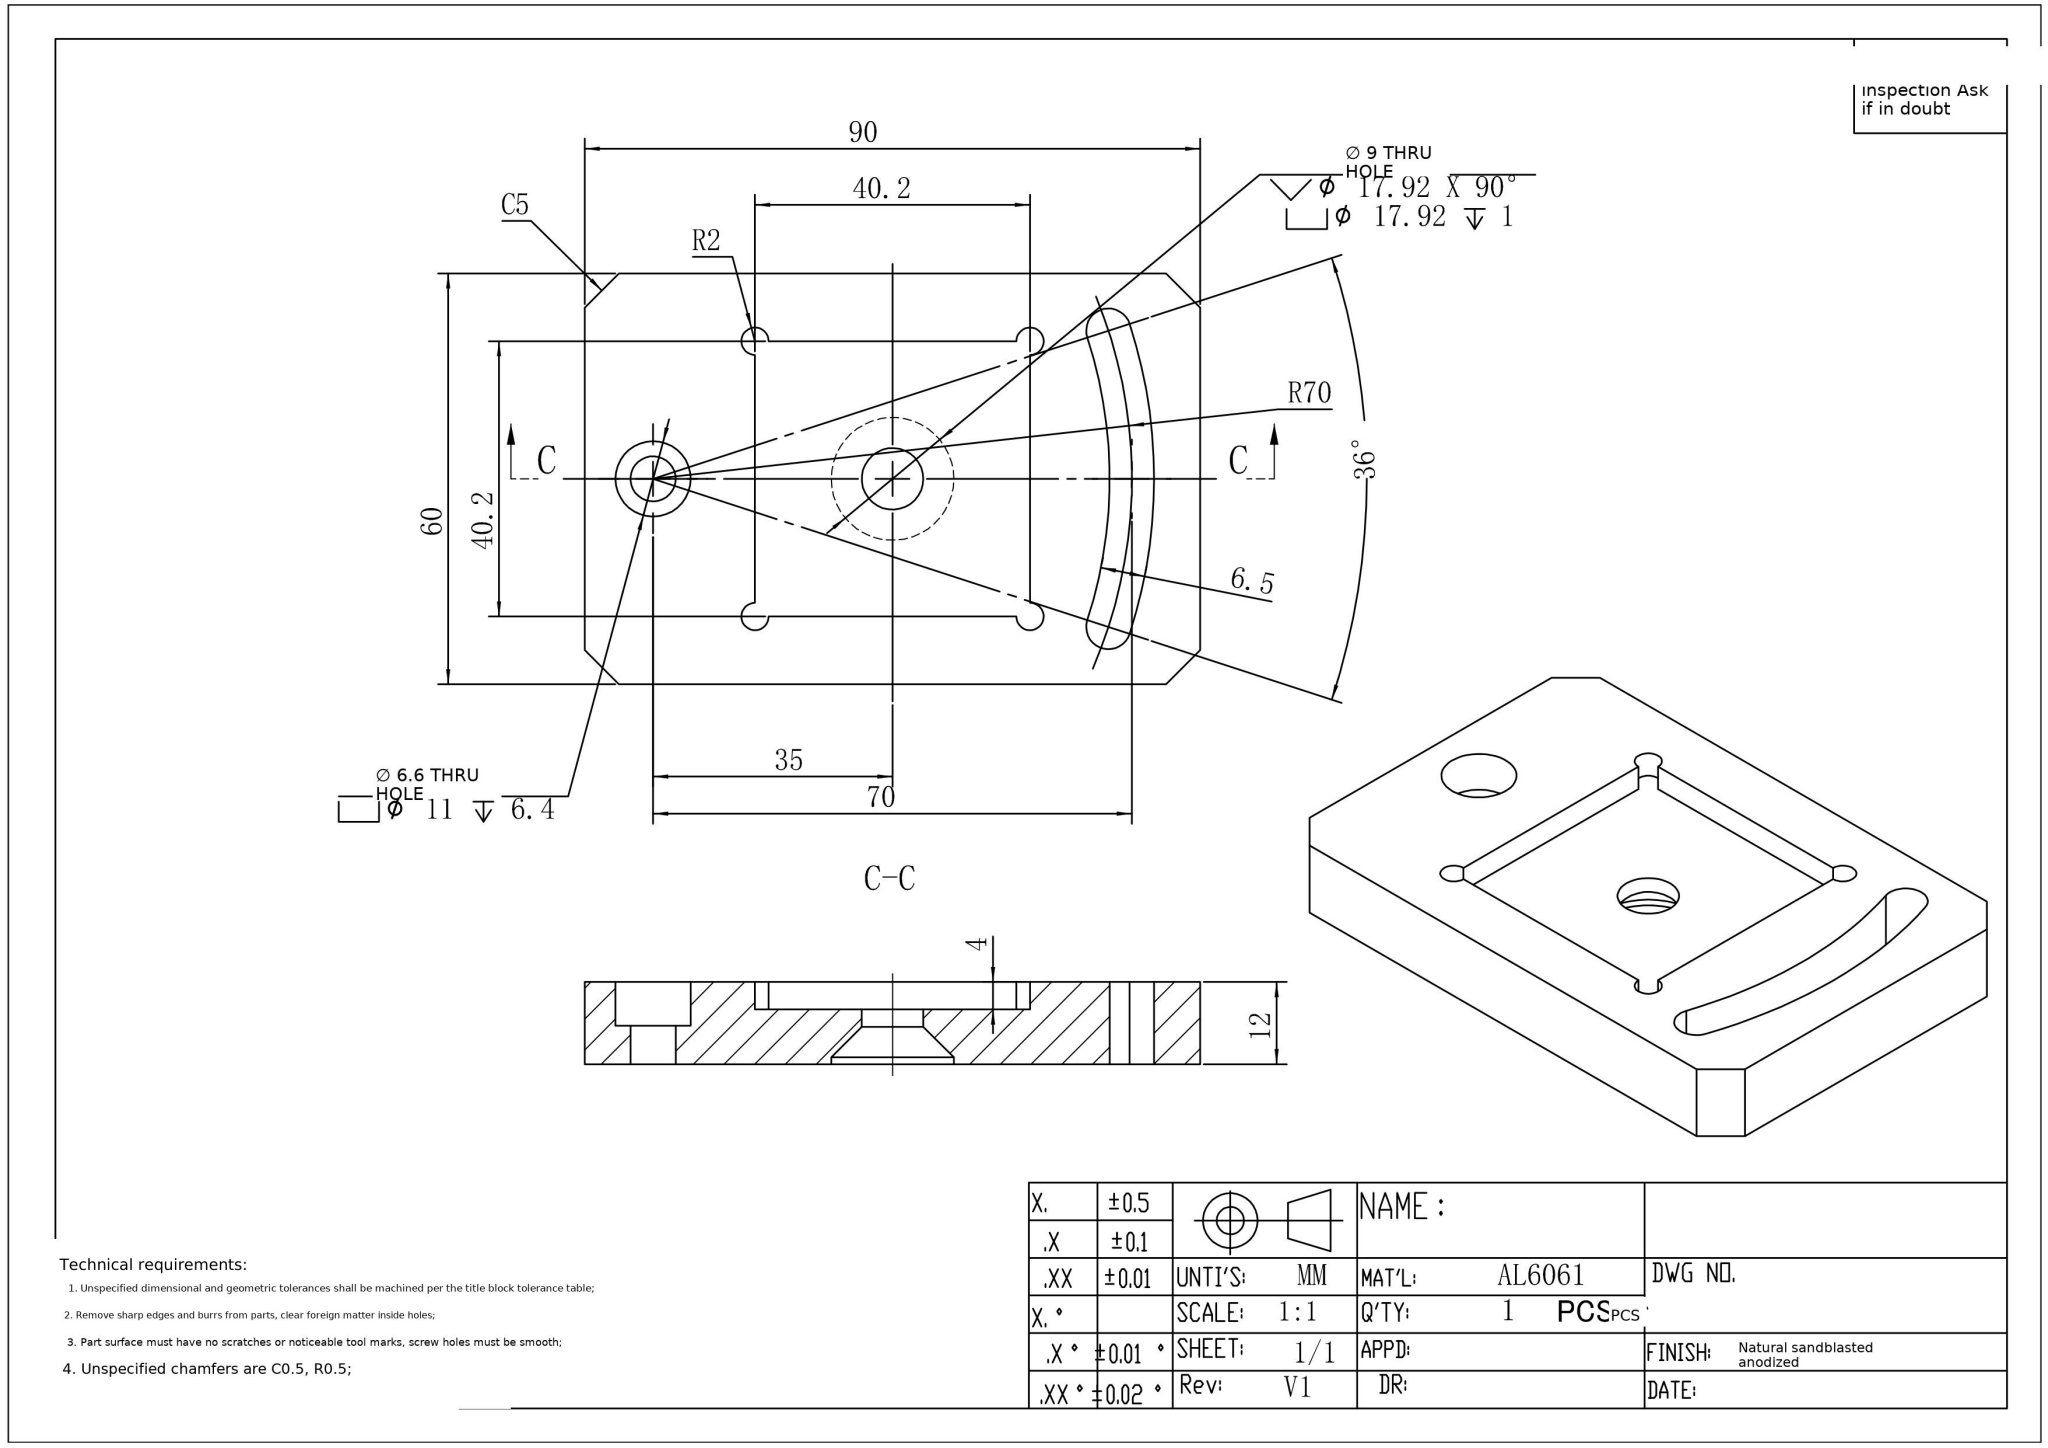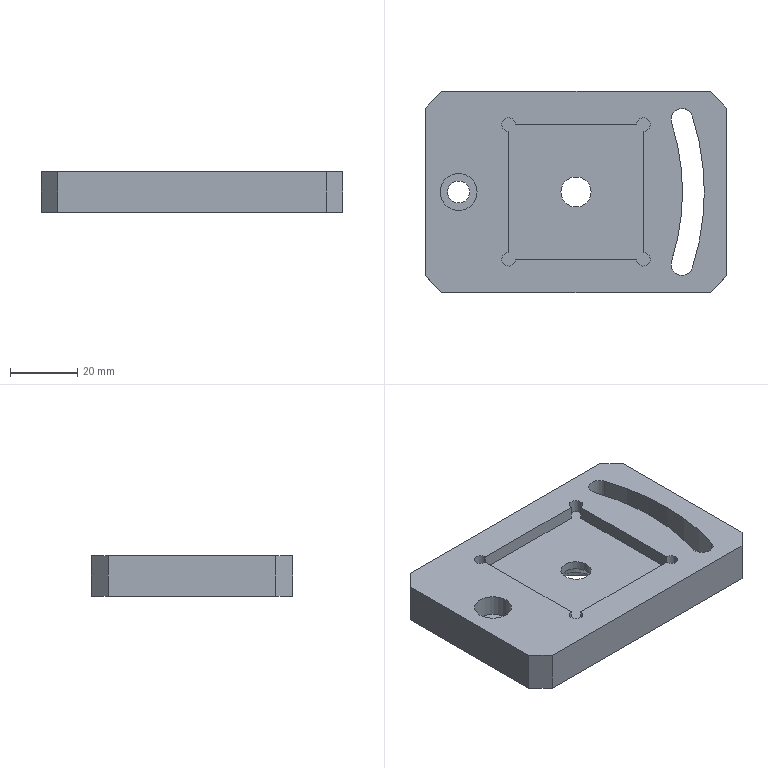Part | NX | mm | 1 solid | 29 faces | box 90 x 60 x 12 mm | volume 51885 mm3 | plane 16 | cylinder 12 | cone 1 | commonest cylinder face diameters 4 x4 6.5 x2 6.6 x1 11 x1 133.5 x1 146.5 x1 17.92 x1 9 x1
STEP:
#1=CARTESIAN_POINT('',(0.,0.,0.));
#2=DIRECTION('',(0.,0.,1.));
#3=DIRECTION('',(1.,0.,0.));
#4=AXIS2_PLACEMENT_3D('',#1,#2,#3);
#5=(LENGTH_UNIT()NAMED_UNIT(*)SI_UNIT(.MILLI.,.METRE.));
#6=UNCERTAINTY_MEASURE_WITH_UNIT(LENGTH_MEASURE(0.00002),#5,'','');
#7=(NAMED_UNIT(*)PLANE_ANGLE_UNIT()SI_UNIT($,.RADIAN.));
#8=PLANE_ANGLE_MEASURE_WITH_UNIT(PLANE_ANGLE_MEASURE(0.01745),#7);
#9=DIMENSIONAL_EXPONENTS(0.,0.,0.,0.,0.,0.,0.);
#10=(CONVERSION_BASED_UNIT('',#8)NAMED_UNIT(#9)PLANE_ANGLE_UNIT());
#11=(NAMED_UNIT(*)SI_UNIT($,.STERADIAN.)SOLID_ANGLE_UNIT());
#12=(GEOMETRIC_REPRESENTATION_CONTEXT(3)GLOBAL_UNCERTAINTY_ASSIGNED_CONTEXT((#6))GLOBAL_UNIT_ASSIGNED_CONTEXT((#5,#10,#11))REPRESENTATION_CONTEXT('',''));
#13=SHAPE_REPRESENTATION('',(#4),#12);
#14=CARTESIAN_POINT('',(85.,60.,0.));
#15=VERTEX_POINT('',#14);
#16=CARTESIAN_POINT('',(5.,60.,0.));
#17=VERTEX_POINT('',#16);
#18=CARTESIAN_POINT('',(90.,60.,0.));
#19=DIRECTION('',(-1.,0.,0.));
#20=VECTOR('',#19,1.);
#21=LINE('',#18,#20);
#22=EDGE_CURVE('',#15,#17,#21,.T.);
#23=ORIENTED_EDGE('',*,*,#22,.F.);
#24=CARTESIAN_POINT('',(85.,60.,-12.));
#25=VERTEX_POINT('',#24);
#26=CARTESIAN_POINT('',(85.,60.,-12.));
#27=DIRECTION('',(0.,0.,-1.));
#28=VECTOR('',#27,1.);
#29=LINE('',#26,#28);
#30=EDGE_CURVE('',#15,#25,#29,.T.);
#31=ORIENTED_EDGE('',*,*,#30,.T.);
#32=CARTESIAN_POINT('',(5.,60.,-12.));
#33=VERTEX_POINT('',#32);
#34=CARTESIAN_POINT('',(90.,60.,-12.));
#35=DIRECTION('',(-1.,0.,0.));
#36=VECTOR('',#35,1.);
#37=LINE('',#34,#36);
#38=EDGE_CURVE('',#25,#33,#37,.T.);
#39=ORIENTED_EDGE('',*,*,#38,.T.);
#40=CARTESIAN_POINT('',(5.,60.,-12.));
#41=DIRECTION('',(0.,0.,1.));
#42=VECTOR('',#41,1.);
#43=LINE('',#40,#42);
#44=EDGE_CURVE('',#33,#17,#43,.T.);
#45=ORIENTED_EDGE('',*,*,#44,.T.);
#46=EDGE_LOOP('',(#23,#31,#39,#45));
#47=FACE_OUTER_BOUND('',#46,.T.);
#48=CARTESIAN_POINT('',(90.,60.,-12.));
#49=DIRECTION('',(0.,1.,0.));
#50=DIRECTION('',(0.,0.,1.));
#51=AXIS2_PLACEMENT_3D('',#48,#49,#50);
#52=PLANE('',#51);
#53=ADVANCED_FACE('',(#47),#52,.T.);
#54=CARTESIAN_POINT('',(0.,55.,-12.));
#55=VERTEX_POINT('',#54);
#56=CARTESIAN_POINT('',(0.,5.,-12.));
#57=VERTEX_POINT('',#56);
#58=CARTESIAN_POINT('',(0.,60.,-12.));
#59=DIRECTION('',(0.,-1.,0.));
#60=VECTOR('',#59,1.);
#61=LINE('',#58,#60);
#62=EDGE_CURVE('',#55,#57,#61,.T.);
#63=ORIENTED_EDGE('',*,*,#62,.T.);
#64=CARTESIAN_POINT('',(0.,5.,0.));
#65=VERTEX_POINT('',#64);
#66=CARTESIAN_POINT('',(0.,5.,-12.));
#67=DIRECTION('',(0.,0.,1.));
#68=VECTOR('',#67,1.);
#69=LINE('',#66,#68);
#70=EDGE_CURVE('',#57,#65,#69,.T.);
#71=ORIENTED_EDGE('',*,*,#70,.T.);
#72=CARTESIAN_POINT('',(0.,55.,0.));
#73=VERTEX_POINT('',#72);
#74=CARTESIAN_POINT('',(0.,60.,0.));
#75=DIRECTION('',(0.,-1.,0.));
#76=VECTOR('',#75,1.);
#77=LINE('',#74,#76);
#78=EDGE_CURVE('',#73,#65,#77,.T.);
#79=ORIENTED_EDGE('',*,*,#78,.F.);
#80=CARTESIAN_POINT('',(0.,55.,-12.));
#81=DIRECTION('',(0.,0.,-1.));
#82=VECTOR('',#81,1.);
#83=LINE('',#80,#82);
#84=EDGE_CURVE('',#73,#55,#83,.T.);
#85=ORIENTED_EDGE('',*,*,#84,.T.);
#86=EDGE_LOOP('',(#63,#71,#79,#85));
#87=FACE_OUTER_BOUND('',#86,.T.);
#88=CARTESIAN_POINT('',(0.,60.,-12.));
#89=DIRECTION('',(-1.,0.,0.));
#90=DIRECTION('',(0.,0.,1.));
#91=AXIS2_PLACEMENT_3D('',#88,#89,#90);
#92=PLANE('',#91);
#93=ADVANCED_FACE('',(#87),#92,.T.);
#94=CARTESIAN_POINT('',(5.,0.,0.));
#95=VERTEX_POINT('',#94);
#96=CARTESIAN_POINT('',(85.,0.,0.));
#97=VERTEX_POINT('',#96);
#98=CARTESIAN_POINT('',(0.,0.,0.));
#99=DIRECTION('',(1.,-0.,0.));
#100=VECTOR('',#99,1.);
#101=LINE('',#98,#100);
#102=EDGE_CURVE('',#95,#97,#101,.T.);
#103=ORIENTED_EDGE('',*,*,#102,.F.);
#104=CARTESIAN_POINT('',(5.,0.,-12.));
#105=VERTEX_POINT('',#104);
#106=CARTESIAN_POINT('',(5.,0.,-12.));
#107=DIRECTION('',(0.,0.,-1.));
#108=VECTOR('',#107,1.);
#109=LINE('',#106,#108);
#110=EDGE_CURVE('',#95,#105,#109,.T.);
#111=ORIENTED_EDGE('',*,*,#110,.T.);
#112=CARTESIAN_POINT('',(85.,0.,-12.));
#113=VERTEX_POINT('',#112);
#114=CARTESIAN_POINT('',(0.,0.,-12.));
#115=DIRECTION('',(1.,-0.,0.));
#116=VECTOR('',#115,1.);
#117=LINE('',#114,#116);
#118=EDGE_CURVE('',#105,#113,#117,.T.);
#119=ORIENTED_EDGE('',*,*,#118,.T.);
#120=CARTESIAN_POINT('',(85.,0.,-12.));
#121=DIRECTION('',(0.,0.,1.));
#122=VECTOR('',#121,1.);
#123=LINE('',#120,#122);
#124=EDGE_CURVE('',#113,#97,#123,.T.);
#125=ORIENTED_EDGE('',*,*,#124,.T.);
#126=EDGE_LOOP('',(#103,#111,#119,#125));
#127=FACE_OUTER_BOUND('',#126,.T.);
#128=CARTESIAN_POINT('',(0.,0.,-12.));
#129=DIRECTION('',(-0.,-1.,0.));
#130=DIRECTION('',(1.,-0.,0.));
#131=AXIS2_PLACEMENT_3D('',#128,#129,#130);
#132=PLANE('',#131);
#133=ADVANCED_FACE('',(#127),#132,.T.);
#134=CARTESIAN_POINT('',(90.,5.,0.));
#135=VERTEX_POINT('',#134);
#136=CARTESIAN_POINT('',(90.,55.,0.));
#137=VERTEX_POINT('',#136);
#138=CARTESIAN_POINT('',(90.,0.,0.));
#139=DIRECTION('',(-0.,1.,0.));
#140=VECTOR('',#139,1.);
#141=LINE('',#138,#140);
#142=EDGE_CURVE('',#135,#137,#141,.T.);
#143=ORIENTED_EDGE('',*,*,#142,.F.);
#144=CARTESIAN_POINT('',(90.,5.,-12.));
#145=VERTEX_POINT('',#144);
#146=CARTESIAN_POINT('',(90.,5.,-12.));
#147=DIRECTION('',(0.,0.,-1.));
#148=VECTOR('',#147,1.);
#149=LINE('',#146,#148);
#150=EDGE_CURVE('',#135,#145,#149,.T.);
#151=ORIENTED_EDGE('',*,*,#150,.T.);
#152=CARTESIAN_POINT('',(90.,55.,-12.));
#153=VERTEX_POINT('',#152);
#154=CARTESIAN_POINT('',(90.,0.,-12.));
#155=DIRECTION('',(-0.,1.,0.));
#156=VECTOR('',#155,1.);
#157=LINE('',#154,#156);
#158=EDGE_CURVE('',#145,#153,#157,.T.);
#159=ORIENTED_EDGE('',*,*,#158,.T.);
#160=CARTESIAN_POINT('',(90.,55.,-12.));
#161=DIRECTION('',(0.,0.,1.));
#162=VECTOR('',#161,1.);
#163=LINE('',#160,#162);
#164=EDGE_CURVE('',#153,#137,#163,.T.);
#165=ORIENTED_EDGE('',*,*,#164,.T.);
#166=EDGE_LOOP('',(#143,#151,#159,#165));
#167=FACE_OUTER_BOUND('',#166,.T.);
#168=CARTESIAN_POINT('',(90.,0.,-12.));
#169=DIRECTION('',(1.,0.,0.));
#170=DIRECTION('',(-0.,1.,0.));
#171=AXIS2_PLACEMENT_3D('',#168,#169,#170);
#172=PLANE('',#171);
#173=ADVANCED_FACE('',(#167),#172,.T.);
#174=CARTESIAN_POINT('',(53.96,30.,-12.));
#175=VERTEX_POINT('',#174);
#176=CARTESIAN_POINT('',(45.,30.,-12.));
#177=DIRECTION('',(0.,0.,1.));
#178=DIRECTION('',(1.,0.,0.));
#179=AXIS2_PLACEMENT_3D('',#176,#177,#178);
#180=CIRCLE('',#179,8.96);
#181=EDGE_CURVE('',#175,#175,#180,.T.);
#182=ORIENTED_EDGE('',*,*,#181,.T.);
#183=EDGE_LOOP('',(#182));
#184=FACE_BOUND('',#183,.T.);
#185=CARTESIAN_POINT('',(79.665,7.365,-12.));
#186=VERTEX_POINT('',#185);
#187=CARTESIAN_POINT('',(73.483,9.373,-12.));
#188=VERTEX_POINT('',#187);
#189=CARTESIAN_POINT('',(76.574,8.369,-12.));
#190=DIRECTION('',(0.,0.,-1.));
#191=DIRECTION('',(1.,0.,0.));
#192=AXIS2_PLACEMENT_3D('',#189,#190,#191);
#193=CIRCLE('',#192,3.25);
#194=EDGE_CURVE('',#186,#188,#193,.T.);
#195=ORIENTED_EDGE('',*,*,#194,.F.);
#196=CARTESIAN_POINT('',(79.665,52.635,-12.));
#197=VERTEX_POINT('',#196);
#198=CARTESIAN_POINT('',(10.,30.,-12.));
#199=DIRECTION('',(0.,0.,-1.));
#200=DIRECTION('',(1.,0.,0.));
#201=AXIS2_PLACEMENT_3D('',#198,#199,#200);
#202=CIRCLE('',#201,73.25);
#203=EDGE_CURVE('',#197,#186,#202,.T.);
#204=ORIENTED_EDGE('',*,*,#203,.F.);
#205=CARTESIAN_POINT('',(73.483,50.627,-12.));
#206=VERTEX_POINT('',#205);
#207=CARTESIAN_POINT('',(76.574,51.631,-12.));
#208=DIRECTION('',(0.,0.,-1.));
#209=DIRECTION('',(1.,0.,0.));
#210=AXIS2_PLACEMENT_3D('',#207,#208,#209);
#211=CIRCLE('',#210,3.25);
#212=EDGE_CURVE('',#206,#197,#211,.T.);
#213=ORIENTED_EDGE('',*,*,#212,.F.);
#214=CARTESIAN_POINT('',(10.,30.,-12.));
#215=DIRECTION('',(0.,0.,1.));
#216=DIRECTION('',(1.,0.,0.));
#217=AXIS2_PLACEMENT_3D('',#214,#215,#216);
#218=CIRCLE('',#217,66.75);
#219=EDGE_CURVE('',#188,#206,#218,.T.);
#220=ORIENTED_EDGE('',*,*,#219,.F.);
#221=EDGE_LOOP('',(#195,#204,#213,#220));
#222=FACE_BOUND('',#221,.T.);
#223=CARTESIAN_POINT('',(13.3,30.,-12.));
#224=VERTEX_POINT('',#223);
#225=CARTESIAN_POINT('',(10.,30.,-12.));
#226=DIRECTION('',(0.,0.,1.));
#227=DIRECTION('',(1.,0.,0.));
#228=AXIS2_PLACEMENT_3D('',#225,#226,#227);
#229=CIRCLE('',#228,3.3);
#230=EDGE_CURVE('',#224,#224,#229,.T.);
#231=ORIENTED_EDGE('',*,*,#230,.T.);
#232=EDGE_LOOP('',(#231));
#233=FACE_BOUND('',#232,.T.);
#234=ORIENTED_EDGE('',*,*,#118,.F.);
#235=CARTESIAN_POINT('',(0.,5.,-12.));
#236=DIRECTION('',(-0.7071,0.7071,0.));
#237=VECTOR('',#236,1.);
#238=LINE('',#235,#237);
#239=EDGE_CURVE('',#105,#57,#238,.T.);
#240=ORIENTED_EDGE('',*,*,#239,.T.);
#241=ORIENTED_EDGE('',*,*,#62,.F.);
#242=CARTESIAN_POINT('',(5.,60.,-12.));
#243=DIRECTION('',(0.7071,0.7071,0.));
#244=VECTOR('',#243,1.);
#245=LINE('',#242,#244);
#246=EDGE_CURVE('',#55,#33,#245,.T.);
#247=ORIENTED_EDGE('',*,*,#246,.T.);
#248=ORIENTED_EDGE('',*,*,#38,.F.);
#249=CARTESIAN_POINT('',(90.,55.,-12.));
#250=DIRECTION('',(0.7071,-0.7071,0.));
#251=VECTOR('',#250,1.);
#252=LINE('',#249,#251);
#253=EDGE_CURVE('',#25,#153,#252,.T.);
#254=ORIENTED_EDGE('',*,*,#253,.T.);
#255=ORIENTED_EDGE('',*,*,#158,.F.);
#256=CARTESIAN_POINT('',(85.,0.,-12.));
#257=DIRECTION('',(-0.7071,-0.7071,0.));
#258=VECTOR('',#257,1.);
#259=LINE('',#256,#258);
#260=EDGE_CURVE('',#145,#113,#259,.T.);
#261=ORIENTED_EDGE('',*,*,#260,.T.);
#262=EDGE_LOOP('',(#234,#240,#241,#247,#248,#254,#255,#261));
#263=FACE_BOUND('',#262,.T.);
#264=CARTESIAN_POINT('',(0.,0.,-12.));
#265=DIRECTION('',(0.,0.,1.));
#266=DIRECTION('',(1.,0.,0.));
#267=AXIS2_PLACEMENT_3D('',#264,#265,#266);
#268=PLANE('',#267);
#269=ADVANCED_FACE('',(#184,#222,#233,#263),#268,.F.);
#270=CARTESIAN_POINT('',(79.665,52.635,0.));
#271=VERTEX_POINT('',#270);
#272=CARTESIAN_POINT('',(79.665,7.365,0.));
#273=VERTEX_POINT('',#272);
#274=CARTESIAN_POINT('',(10.,30.,0.));
#275=DIRECTION('',(0.,0.,-1.));
#276=DIRECTION('',(1.,0.,0.));
#277=AXIS2_PLACEMENT_3D('',#274,#275,#276);
#278=CIRCLE('',#277,73.25);
#279=EDGE_CURVE('',#271,#273,#278,.T.);
#280=ORIENTED_EDGE('',*,*,#279,.T.);
#281=CARTESIAN_POINT('',(73.483,9.373,0.));
#282=VERTEX_POINT('',#281);
#283=CARTESIAN_POINT('',(76.574,8.369,0.));
#284=DIRECTION('',(0.,0.,-1.));
#285=DIRECTION('',(1.,0.,0.));
#286=AXIS2_PLACEMENT_3D('',#283,#284,#285);
#287=CIRCLE('',#286,3.25);
#288=EDGE_CURVE('',#273,#282,#287,.T.);
#289=ORIENTED_EDGE('',*,*,#288,.T.);
#290=CARTESIAN_POINT('',(73.483,50.627,0.));
#291=VERTEX_POINT('',#290);
#292=CARTESIAN_POINT('',(10.,30.,0.));
#293=DIRECTION('',(0.,0.,1.));
#294=DIRECTION('',(1.,0.,0.));
#295=AXIS2_PLACEMENT_3D('',#292,#293,#294);
#296=CIRCLE('',#295,66.75);
#297=EDGE_CURVE('',#282,#291,#296,.T.);
#298=ORIENTED_EDGE('',*,*,#297,.T.);
#299=CARTESIAN_POINT('',(76.574,51.631,0.));
#300=DIRECTION('',(0.,0.,-1.));
#301=DIRECTION('',(1.,0.,0.));
#302=AXIS2_PLACEMENT_3D('',#299,#300,#301);
#303=CIRCLE('',#302,3.25);
#304=EDGE_CURVE('',#291,#271,#303,.T.);
#305=ORIENTED_EDGE('',*,*,#304,.T.);
#306=EDGE_LOOP('',(#280,#289,#298,#305));
#307=FACE_BOUND('',#306,.T.);
#308=CARTESIAN_POINT('',(65.1,11.9,0.));
#309=VERTEX_POINT('',#308);
#310=CARTESIAN_POINT('',(65.1,48.1,0.));
#311=VERTEX_POINT('',#310);
#312=CARTESIAN_POINT('',(65.1,11.9,0.));
#313=DIRECTION('',(0.,1.,0.));
#314=VECTOR('',#313,1.);
#315=LINE('',#312,#314);
#316=EDGE_CURVE('',#309,#311,#315,.T.);
#317=ORIENTED_EDGE('',*,*,#316,.F.);
#318=CARTESIAN_POINT('',(63.1,9.9,0.));
#319=VERTEX_POINT('',#318);
#320=CARTESIAN_POINT('',(65.1,9.9,0.));
#321=DIRECTION('',(0.,0.,1.));
#322=DIRECTION('',(1.,0.,0.));
#323=AXIS2_PLACEMENT_3D('',#320,#321,#322);
#324=CIRCLE('',#323,2.);
#325=EDGE_CURVE('',#319,#309,#324,.T.);
#326=ORIENTED_EDGE('',*,*,#325,.F.);
#327=CARTESIAN_POINT('',(26.9,9.9,0.));
#328=VERTEX_POINT('',#327);
#329=CARTESIAN_POINT('',(26.9,9.9,0.));
#330=DIRECTION('',(1.,0.,0.));
#331=VECTOR('',#330,1.);
#332=LINE('',#329,#331);
#333=EDGE_CURVE('',#328,#319,#332,.T.);
#334=ORIENTED_EDGE('',*,*,#333,.F.);
#335=CARTESIAN_POINT('',(24.9,11.9,0.));
#336=VERTEX_POINT('',#335);
#337=CARTESIAN_POINT('',(24.9,9.9,0.));
#338=DIRECTION('',(0.,0.,1.));
#339=DIRECTION('',(1.,0.,0.));
#340=AXIS2_PLACEMENT_3D('',#337,#338,#339);
#341=CIRCLE('',#340,2.);
#342=EDGE_CURVE('',#336,#328,#341,.T.);
#343=ORIENTED_EDGE('',*,*,#342,.F.);
#344=CARTESIAN_POINT('',(24.9,48.1,0.));
#345=VERTEX_POINT('',#344);
#346=CARTESIAN_POINT('',(24.9,48.1,0.));
#347=DIRECTION('',(0.,-1.,0.));
#348=VECTOR('',#347,1.);
#349=LINE('',#346,#348);
#350=EDGE_CURVE('',#345,#336,#349,.T.);
#351=ORIENTED_EDGE('',*,*,#350,.F.);
#352=CARTESIAN_POINT('',(26.9,50.1,0.));
#353=VERTEX_POINT('',#352);
#354=CARTESIAN_POINT('',(24.9,50.1,0.));
#355=DIRECTION('',(0.,0.,1.));
#356=DIRECTION('',(1.,0.,0.));
#357=AXIS2_PLACEMENT_3D('',#354,#355,#356);
#358=CIRCLE('',#357,2.);
#359=EDGE_CURVE('',#353,#345,#358,.T.);
#360=ORIENTED_EDGE('',*,*,#359,.F.);
#361=CARTESIAN_POINT('',(63.1,50.1,0.));
#362=VERTEX_POINT('',#361);
#363=CARTESIAN_POINT('',(63.1,50.1,0.));
#364=DIRECTION('',(-1.,0.,0.));
#365=VECTOR('',#364,1.);
#366=LINE('',#363,#365);
#367=EDGE_CURVE('',#362,#353,#366,.T.);
#368=ORIENTED_EDGE('',*,*,#367,.F.);
#369=CARTESIAN_POINT('',(65.1,50.1,0.));
#370=DIRECTION('',(0.,0.,1.));
#371=DIRECTION('',(1.,0.,0.));
#372=AXIS2_PLACEMENT_3D('',#369,#370,#371);
#373=CIRCLE('',#372,2.);
#374=EDGE_CURVE('',#311,#362,#373,.T.);
#375=ORIENTED_EDGE('',*,*,#374,.F.);
#376=EDGE_LOOP('',(#317,#326,#334,#343,#351,#360,#368,#375));
#377=FACE_BOUND('',#376,.T.);
#378=CARTESIAN_POINT('',(15.5,30.,0.));
#379=VERTEX_POINT('',#378);
#380=CARTESIAN_POINT('',(10.,30.,0.));
#381=DIRECTION('',(0.,0.,-1.));
#382=DIRECTION('',(1.,0.,0.));
#383=AXIS2_PLACEMENT_3D('',#380,#381,#382);
#384=CIRCLE('',#383,5.5);
#385=EDGE_CURVE('',#379,#379,#384,.T.);
#386=ORIENTED_EDGE('',*,*,#385,.T.);
#387=EDGE_LOOP('',(#386));
#388=FACE_BOUND('',#387,.T.);
#389=ORIENTED_EDGE('',*,*,#78,.T.);
#390=CARTESIAN_POINT('',(2.5,2.5,0.));
#391=DIRECTION('',(0.7071,-0.7071,0.));
#392=VECTOR('',#391,1.);
#393=LINE('',#390,#392);
#394=EDGE_CURVE('',#65,#95,#393,.T.);
#395=ORIENTED_EDGE('',*,*,#394,.T.);
#396=ORIENTED_EDGE('',*,*,#102,.T.);
#397=CARTESIAN_POINT('',(42.5,-42.5,0.));
#398=DIRECTION('',(0.7071,0.7071,0.));
#399=VECTOR('',#398,1.);
#400=LINE('',#397,#399);
#401=EDGE_CURVE('',#97,#135,#400,.T.);
#402=ORIENTED_EDGE('',*,*,#401,.T.);
#403=ORIENTED_EDGE('',*,*,#142,.T.);
#404=CARTESIAN_POINT('',(72.5,72.5,0.));
#405=DIRECTION('',(-0.7071,0.7071,0.));
#406=VECTOR('',#405,1.);
#407=LINE('',#404,#406);
#408=EDGE_CURVE('',#137,#15,#407,.T.);
#409=ORIENTED_EDGE('',*,*,#408,.T.);
#410=ORIENTED_EDGE('',*,*,#22,.T.);
#411=CARTESIAN_POINT('',(-27.5,27.5,0.));
#412=DIRECTION('',(-0.7071,-0.7071,0.));
#413=VECTOR('',#412,1.);
#414=LINE('',#411,#413);
#415=EDGE_CURVE('',#17,#73,#414,.T.);
#416=ORIENTED_EDGE('',*,*,#415,.T.);
#417=EDGE_LOOP('',(#389,#395,#396,#402,#403,#409,#410,#416));
#418=FACE_BOUND('',#417,.T.);
#419=CARTESIAN_POINT('',(0.,0.,0.));
#420=DIRECTION('',(0.,0.,1.));
#421=DIRECTION('',(1.,0.,0.));
#422=AXIS2_PLACEMENT_3D('',#419,#420,#421);
#423=PLANE('',#422);
#424=ADVANCED_FACE('',(#307,#377,#388,#418),#423,.T.);
#425=CARTESIAN_POINT('',(6.7,30.,-6.4));
#426=VERTEX_POINT('',#425);
#427=CARTESIAN_POINT('',(10.,30.,-6.4));
#428=DIRECTION('',(0.,0.,1.));
#429=DIRECTION('',(-1.,0.,0.));
#430=AXIS2_PLACEMENT_3D('',#427,#428,#429);
#431=CIRCLE('',#430,3.3);
#432=EDGE_CURVE('',#426,#426,#431,.T.);
#433=ORIENTED_EDGE('',*,*,#432,.T.);
#434=EDGE_LOOP('',(#433));
#435=FACE_BOUND('',#434,.T.);
#436=ORIENTED_EDGE('',*,*,#230,.F.);
#437=EDGE_LOOP('',(#436));
#438=FACE_BOUND('',#437,.T.);
#439=CARTESIAN_POINT('',(10.,30.,-12.));
#440=DIRECTION('',(0.,0.,1.));
#441=DIRECTION('',(1.,0.,0.));
#442=AXIS2_PLACEMENT_3D('',#439,#440,#441);
#443=CYLINDRICAL_SURFACE('',#442,3.3);
#444=ADVANCED_FACE('',(#435,#438),#443,.F.);
#445=CARTESIAN_POINT('',(15.5,30.,-6.4));
#446=VERTEX_POINT('',#445);
#447=CARTESIAN_POINT('',(10.,30.,-6.4));
#448=DIRECTION('',(0.,0.,1.));
#449=DIRECTION('',(1.,0.,0.));
#450=AXIS2_PLACEMENT_3D('',#447,#448,#449);
#451=CIRCLE('',#450,5.5);
#452=EDGE_CURVE('',#446,#446,#451,.T.);
#453=ORIENTED_EDGE('',*,*,#452,.T.);
#454=EDGE_LOOP('',(#453));
#455=FACE_BOUND('',#454,.T.);
#456=ORIENTED_EDGE('',*,*,#432,.F.);
#457=EDGE_LOOP('',(#456));
#458=FACE_BOUND('',#457,.T.);
#459=CARTESIAN_POINT('',(10.,30.,-6.4));
#460=DIRECTION('',(0.,0.,-1.));
#461=DIRECTION('',(-1.,0.,0.));
#462=AXIS2_PLACEMENT_3D('',#459,#460,#461);
#463=PLANE('',#462);
#464=ADVANCED_FACE('',(#455,#458),#463,.F.);
#465=ORIENTED_EDGE('',*,*,#452,.F.);
#466=EDGE_LOOP('',(#465));
#467=FACE_BOUND('',#466,.T.);
#468=ORIENTED_EDGE('',*,*,#385,.F.);
#469=EDGE_LOOP('',(#468));
#470=FACE_BOUND('',#469,.T.);
#471=CARTESIAN_POINT('',(10.,30.,-6.4));
#472=DIRECTION('',(0.,0.,1.));
#473=DIRECTION('',(1.,0.,0.));
#474=AXIS2_PLACEMENT_3D('',#471,#472,#473);
#475=CYLINDRICAL_SURFACE('',#474,5.5);
#476=ADVANCED_FACE('',(#467,#470),#475,.F.);
#477=ORIENTED_EDGE('',*,*,#316,.T.);
#478=CARTESIAN_POINT('',(65.1,48.1,-4.));
#479=VERTEX_POINT('',#478);
#480=CARTESIAN_POINT('',(65.1,48.1,-4.));
#481=DIRECTION('',(0.,0.,-1.));
#482=VECTOR('',#481,1.);
#483=LINE('',#480,#482);
#484=EDGE_CURVE('',#311,#479,#483,.T.);
#485=ORIENTED_EDGE('',*,*,#484,.T.);
#486=CARTESIAN_POINT('',(65.1,11.9,-4.));
#487=VERTEX_POINT('',#486);
#488=CARTESIAN_POINT('',(65.1,11.9,-4.));
#489=DIRECTION('',(0.,-1.,0.));
#490=VECTOR('',#489,1.);
#491=LINE('',#488,#490);
#492=EDGE_CURVE('',#479,#487,#491,.T.);
#493=ORIENTED_EDGE('',*,*,#492,.T.);
#494=CARTESIAN_POINT('',(65.1,11.9,-4.));
#495=DIRECTION('',(0.,0.,-1.));
#496=VECTOR('',#495,1.);
#497=LINE('',#494,#496);
#498=EDGE_CURVE('',#309,#487,#497,.T.);
#499=ORIENTED_EDGE('',*,*,#498,.F.);
#500=EDGE_LOOP('',(#477,#485,#493,#499));
#501=FACE_OUTER_BOUND('',#500,.T.);
#502=CARTESIAN_POINT('',(65.1,11.9,-4.));
#503=DIRECTION('',(1.,0.,0.));
#504=DIRECTION('',(0.,0.,-1.));
#505=AXIS2_PLACEMENT_3D('',#502,#503,#504);
#506=PLANE('',#505);
#507=ADVANCED_FACE('',(#501),#506,.F.);
#508=ORIENTED_EDGE('',*,*,#374,.T.);
#509=CARTESIAN_POINT('',(63.1,50.1,-4.));
#510=VERTEX_POINT('',#509);
#511=CARTESIAN_POINT('',(63.1,50.1,-4.));
#512=DIRECTION('',(0.,0.,-1.));
#513=VECTOR('',#512,1.);
#514=LINE('',#511,#513);
#515=EDGE_CURVE('',#362,#510,#514,.T.);
#516=ORIENTED_EDGE('',*,*,#515,.T.);
#517=CARTESIAN_POINT('',(65.1,50.1,-4.));
#518=DIRECTION('',(0.,0.,-1.));
#519=DIRECTION('',(1.,0.,0.));
#520=AXIS2_PLACEMENT_3D('',#517,#518,#519);
#521=CIRCLE('',#520,2.);
#522=EDGE_CURVE('',#510,#479,#521,.T.);
#523=ORIENTED_EDGE('',*,*,#522,.T.);
#524=ORIENTED_EDGE('',*,*,#484,.F.);
#525=EDGE_LOOP('',(#508,#516,#523,#524));
#526=FACE_OUTER_BOUND('',#525,.T.);
#527=CARTESIAN_POINT('',(65.1,50.1,-4.));
#528=DIRECTION('',(0.,0.,1.));
#529=DIRECTION('',(1.,0.,0.));
#530=AXIS2_PLACEMENT_3D('',#527,#528,#529);
#531=CYLINDRICAL_SURFACE('',#530,2.);
#532=ADVANCED_FACE('',(#526),#531,.F.);
#533=ORIENTED_EDGE('',*,*,#367,.T.);
#534=CARTESIAN_POINT('',(26.9,50.1,-4.));
#535=VERTEX_POINT('',#534);
#536=CARTESIAN_POINT('',(26.9,50.1,-4.));
#537=DIRECTION('',(0.,0.,-1.));
#538=VECTOR('',#537,1.);
#539=LINE('',#536,#538);
#540=EDGE_CURVE('',#353,#535,#539,.T.);
#541=ORIENTED_EDGE('',*,*,#540,.T.);
#542=CARTESIAN_POINT('',(63.1,50.1,-4.));
#543=DIRECTION('',(1.,0.,0.));
#544=VECTOR('',#543,1.);
#545=LINE('',#542,#544);
#546=EDGE_CURVE('',#535,#510,#545,.T.);
#547=ORIENTED_EDGE('',*,*,#546,.T.);
#548=ORIENTED_EDGE('',*,*,#515,.F.);
#549=EDGE_LOOP('',(#533,#541,#547,#548));
#550=FACE_OUTER_BOUND('',#549,.T.);
#551=CARTESIAN_POINT('',(63.1,50.1,-4.));
#552=DIRECTION('',(0.,1.,0.));
#553=DIRECTION('',(0.,0.,1.));
#554=AXIS2_PLACEMENT_3D('',#551,#552,#553);
#555=PLANE('',#554);
#556=ADVANCED_FACE('',(#550),#555,.F.);
#557=ORIENTED_EDGE('',*,*,#359,.T.);
#558=CARTESIAN_POINT('',(24.9,48.1,-4.));
#559=VERTEX_POINT('',#558);
#560=CARTESIAN_POINT('',(24.9,48.1,-4.));
#561=DIRECTION('',(0.,0.,-1.));
#562=VECTOR('',#561,1.);
#563=LINE('',#560,#562);
#564=EDGE_CURVE('',#345,#559,#563,.T.);
#565=ORIENTED_EDGE('',*,*,#564,.T.);
#566=CARTESIAN_POINT('',(24.9,50.1,-4.));
#567=DIRECTION('',(0.,0.,-1.));
#568=DIRECTION('',(1.,0.,0.));
#569=AXIS2_PLACEMENT_3D('',#566,#567,#568);
#570=CIRCLE('',#569,2.);
#571=EDGE_CURVE('',#559,#535,#570,.T.);
#572=ORIENTED_EDGE('',*,*,#571,.T.);
#573=ORIENTED_EDGE('',*,*,#540,.F.);
#574=EDGE_LOOP('',(#557,#565,#572,#573));
#575=FACE_OUTER_BOUND('',#574,.T.);
#576=CARTESIAN_POINT('',(24.9,50.1,-4.));
#577=DIRECTION('',(0.,0.,1.));
#578=DIRECTION('',(1.,0.,0.));
#579=AXIS2_PLACEMENT_3D('',#576,#577,#578);
#580=CYLINDRICAL_SURFACE('',#579,2.);
#581=ADVANCED_FACE('',(#575),#580,.F.);
#582=ORIENTED_EDGE('',*,*,#350,.T.);
#583=CARTESIAN_POINT('',(24.9,11.9,-4.));
#584=VERTEX_POINT('',#583);
#585=CARTESIAN_POINT('',(24.9,11.9,-4.));
#586=DIRECTION('',(0.,0.,-1.));
#587=VECTOR('',#586,1.);
#588=LINE('',#585,#587);
#589=EDGE_CURVE('',#336,#584,#588,.T.);
#590=ORIENTED_EDGE('',*,*,#589,.T.);
#591=CARTESIAN_POINT('',(24.9,48.1,-4.));
#592=DIRECTION('',(0.,1.,0.));
#593=VECTOR('',#592,1.);
#594=LINE('',#591,#593);
#595=EDGE_CURVE('',#584,#559,#594,.T.);
#596=ORIENTED_EDGE('',*,*,#595,.T.);
#597=ORIENTED_EDGE('',*,*,#564,.F.);
#598=EDGE_LOOP('',(#582,#590,#596,#597));
#599=FACE_OUTER_BOUND('',#598,.T.);
#600=CARTESIAN_POINT('',(24.9,48.1,-4.));
#601=DIRECTION('',(-1.,0.,0.));
#602=DIRECTION('',(0.,0.,1.));
#603=AXIS2_PLACEMENT_3D('',#600,#601,#602);
#604=PLANE('',#603);
#605=ADVANCED_FACE('',(#599),#604,.F.);
#606=ORIENTED_EDGE('',*,*,#342,.T.);
#607=CARTESIAN_POINT('',(26.9,9.9,-4.));
#608=VERTEX_POINT('',#607);
#609=CARTESIAN_POINT('',(26.9,9.9,-4.));
#610=DIRECTION('',(0.,0.,-1.));
#611=VECTOR('',#610,1.);
#612=LINE('',#609,#611);
#613=EDGE_CURVE('',#328,#608,#612,.T.);
#614=ORIENTED_EDGE('',*,*,#613,.T.);
#615=CARTESIAN_POINT('',(24.9,9.9,-4.));
#616=DIRECTION('',(0.,0.,-1.));
#617=DIRECTION('',(1.,0.,0.));
#618=AXIS2_PLACEMENT_3D('',#615,#616,#617);
#619=CIRCLE('',#618,2.);
#620=EDGE_CURVE('',#608,#584,#619,.T.);
#621=ORIENTED_EDGE('',*,*,#620,.T.);
#622=ORIENTED_EDGE('',*,*,#589,.F.);
#623=EDGE_LOOP('',(#606,#614,#621,#622));
#624=FACE_OUTER_BOUND('',#623,.T.);
#625=CARTESIAN_POINT('',(24.9,9.9,-4.));
#626=DIRECTION('',(0.,0.,1.));
#627=DIRECTION('',(1.,0.,0.));
#628=AXIS2_PLACEMENT_3D('',#625,#626,#627);
#629=CYLINDRICAL_SURFACE('',#628,2.);
#630=ADVANCED_FACE('',(#624),#629,.F.);
#631=ORIENTED_EDGE('',*,*,#333,.T.);
#632=CARTESIAN_POINT('',(63.1,9.9,-4.));
#633=VERTEX_POINT('',#632);
#634=CARTESIAN_POINT('',(63.1,9.9,-4.));
#635=DIRECTION('',(0.,0.,-1.));
#636=VECTOR('',#635,1.);
#637=LINE('',#634,#636);
#638=EDGE_CURVE('',#319,#633,#637,.T.);
#639=ORIENTED_EDGE('',*,*,#638,.T.);
#640=CARTESIAN_POINT('',(26.9,9.9,-4.));
#641=DIRECTION('',(-1.,0.,0.));
#642=VECTOR('',#641,1.);
#643=LINE('',#640,#642);
#644=EDGE_CURVE('',#633,#608,#643,.T.);
#645=ORIENTED_EDGE('',*,*,#644,.T.);
#646=ORIENTED_EDGE('',*,*,#613,.F.);
#647=EDGE_LOOP('',(#631,#639,#645,#646));
#648=FACE_OUTER_BOUND('',#647,.T.);
#649=CARTESIAN_POINT('',(26.9,9.9,-4.));
#650=DIRECTION('',(0.,-1.,0.));
#651=DIRECTION('',(0.,0.,-1.));
#652=AXIS2_PLACEMENT_3D('',#649,#650,#651);
#653=PLANE('',#652);
#654=ADVANCED_FACE('',(#648),#653,.F.);
#655=ORIENTED_EDGE('',*,*,#325,.T.);
#656=ORIENTED_EDGE('',*,*,#498,.T.);
#657=CARTESIAN_POINT('',(65.1,9.9,-4.));
#658=DIRECTION('',(0.,0.,-1.));
#659=DIRECTION('',(1.,0.,0.));
#660=AXIS2_PLACEMENT_3D('',#657,#658,#659);
#661=CIRCLE('',#660,2.);
#662=EDGE_CURVE('',#487,#633,#661,.T.);
#663=ORIENTED_EDGE('',*,*,#662,.T.);
#664=ORIENTED_EDGE('',*,*,#638,.F.);
#665=EDGE_LOOP('',(#655,#656,#663,#664));
#666=FACE_OUTER_BOUND('',#665,.T.);
#667=CARTESIAN_POINT('',(65.1,9.9,-4.));
#668=DIRECTION('',(0.,0.,1.));
#669=DIRECTION('',(1.,0.,0.));
#670=AXIS2_PLACEMENT_3D('',#667,#668,#669);
#671=CYLINDRICAL_SURFACE('',#670,2.);
#672=ADVANCED_FACE('',(#666),#671,.F.);
#673=CARTESIAN_POINT('',(49.5,30.,-4.));
#674=VERTEX_POINT('',#673);
#675=CARTESIAN_POINT('',(45.,30.,-4.));
#676=DIRECTION('',(0.,0.,1.));
#677=DIRECTION('',(1.,0.,0.));
#678=AXIS2_PLACEMENT_3D('',#675,#676,#677);
#679=CIRCLE('',#678,4.5);
#680=EDGE_CURVE('',#674,#674,#679,.T.);
#681=ORIENTED_EDGE('',*,*,#680,.F.);
#682=EDGE_LOOP('',(#681));
#683=FACE_BOUND('',#682,.T.);
#684=ORIENTED_EDGE('',*,*,#492,.F.);
#685=ORIENTED_EDGE('',*,*,#522,.F.);
#686=ORIENTED_EDGE('',*,*,#546,.F.);
#687=ORIENTED_EDGE('',*,*,#571,.F.);
#688=ORIENTED_EDGE('',*,*,#595,.F.);
#689=ORIENTED_EDGE('',*,*,#620,.F.);
#690=ORIENTED_EDGE('',*,*,#644,.F.);
#691=ORIENTED_EDGE('',*,*,#662,.F.);
#692=EDGE_LOOP('',(#684,#685,#686,#687,#688,#689,#690,#691));
#693=FACE_BOUND('',#692,.T.);
#694=CARTESIAN_POINT('',(65.1,50.1,-4.));
#695=DIRECTION('',(0.,0.,1.));
#696=DIRECTION('',(1.,0.,0.));
#697=AXIS2_PLACEMENT_3D('',#694,#695,#696);
#698=PLANE('',#697);
#699=ADVANCED_FACE('',(#683,#693),#698,.T.);
#700=ORIENTED_EDGE('',*,*,#288,.F.);
#701=CARTESIAN_POINT('',(79.665,7.365,-12.));
#702=DIRECTION('',(0.,0.,-1.));
#703=VECTOR('',#702,1.);
#704=LINE('',#701,#703);
#705=EDGE_CURVE('',#273,#186,#704,.T.);
#706=ORIENTED_EDGE('',*,*,#705,.T.);
#707=ORIENTED_EDGE('',*,*,#194,.T.);
#708=CARTESIAN_POINT('',(73.483,9.373,-12.));
#709=DIRECTION('',(0.,0.,-1.));
#710=VECTOR('',#709,1.);
#711=LINE('',#708,#710);
#712=EDGE_CURVE('',#282,#188,#711,.T.);
#713=ORIENTED_EDGE('',*,*,#712,.F.);
#714=EDGE_LOOP('',(#700,#706,#707,#713));
#715=FACE_OUTER_BOUND('',#714,.T.);
#716=CARTESIAN_POINT('',(76.574,8.369,-12.));
#717=DIRECTION('',(0.,0.,1.));
#718=DIRECTION('',(1.,0.,0.));
#719=AXIS2_PLACEMENT_3D('',#716,#717,#718);
#720=CYLINDRICAL_SURFACE('',#719,3.25);
#721=ADVANCED_FACE('',(#715),#720,.F.);
#722=ORIENTED_EDGE('',*,*,#297,.F.);
#723=ORIENTED_EDGE('',*,*,#712,.T.);
#724=ORIENTED_EDGE('',*,*,#219,.T.);
#725=CARTESIAN_POINT('',(73.483,50.627,-12.));
#726=DIRECTION('',(0.,0.,-1.));
#727=VECTOR('',#726,1.);
#728=LINE('',#725,#727);
#729=EDGE_CURVE('',#291,#206,#728,.T.);
#730=ORIENTED_EDGE('',*,*,#729,.F.);
#731=EDGE_LOOP('',(#722,#723,#724,#730));
#732=FACE_OUTER_BOUND('',#731,.T.);
#733=CARTESIAN_POINT('',(10.,30.,-12.));
#734=DIRECTION('',(0.,0.,1.));
#735=DIRECTION('',(1.,0.,0.));
#736=AXIS2_PLACEMENT_3D('',#733,#734,#735);
#737=CYLINDRICAL_SURFACE('',#736,66.75);
#738=ADVANCED_FACE('',(#732),#737,.T.);
#739=ORIENTED_EDGE('',*,*,#304,.F.);
#740=ORIENTED_EDGE('',*,*,#729,.T.);
#741=ORIENTED_EDGE('',*,*,#212,.T.);
#742=CARTESIAN_POINT('',(79.665,52.635,-12.));
#743=DIRECTION('',(0.,0.,-1.));
#744=VECTOR('',#743,1.);
#745=LINE('',#742,#744);
#746=EDGE_CURVE('',#271,#197,#745,.T.);
#747=ORIENTED_EDGE('',*,*,#746,.F.);
#748=EDGE_LOOP('',(#739,#740,#741,#747));
#749=FACE_OUTER_BOUND('',#748,.T.);
#750=CARTESIAN_POINT('',(76.574,51.631,-12.));
#751=DIRECTION('',(0.,0.,1.));
#752=DIRECTION('',(1.,0.,0.));
#753=AXIS2_PLACEMENT_3D('',#750,#751,#752);
#754=CYLINDRICAL_SURFACE('',#753,3.25);
#755=ADVANCED_FACE('',(#749),#754,.F.);
#756=ORIENTED_EDGE('',*,*,#279,.F.);
#757=ORIENTED_EDGE('',*,*,#746,.T.);
#758=ORIENTED_EDGE('',*,*,#203,.T.);
#759=ORIENTED_EDGE('',*,*,#705,.F.);
#760=EDGE_LOOP('',(#756,#757,#758,#759));
#761=FACE_OUTER_BOUND('',#760,.T.);
#762=CARTESIAN_POINT('',(10.,30.,-12.));
#763=DIRECTION('',(0.,0.,1.));
#764=DIRECTION('',(1.,0.,0.));
#765=AXIS2_PLACEMENT_3D('',#762,#763,#764);
#766=CYLINDRICAL_SURFACE('',#765,73.25);
#767=ADVANCED_FACE('',(#761),#766,.F.);
#768=ORIENTED_EDGE('',*,*,#181,.F.);
#769=EDGE_LOOP('',(#768));
#770=FACE_BOUND('',#769,.T.);
#771=CARTESIAN_POINT('',(53.96,30.,-11.));
#772=VERTEX_POINT('',#771);
#773=CARTESIAN_POINT('',(45.,30.,-11.));
#774=DIRECTION('',(0.,0.,-1.));
#775=DIRECTION('',(1.,0.,0.));
#776=AXIS2_PLACEMENT_3D('',#773,#774,#775);
#777=CIRCLE('',#776,8.96);
#778=EDGE_CURVE('',#772,#772,#777,.T.);
#779=ORIENTED_EDGE('',*,*,#778,.F.);
#780=EDGE_LOOP('',(#779));
#781=FACE_BOUND('',#780,.T.);
#782=CARTESIAN_POINT('',(45.,30.,0.));
#783=DIRECTION('',(0.,0.,1.));
#784=DIRECTION('',(1.,0.,0.));
#785=AXIS2_PLACEMENT_3D('',#782,#783,#784);
#786=CYLINDRICAL_SURFACE('',#785,8.96);
#787=ADVANCED_FACE('',(#770,#781),#786,.F.);
#788=ORIENTED_EDGE('',*,*,#778,.T.);
#789=EDGE_LOOP('',(#788));
#790=FACE_BOUND('',#789,.T.);
#791=CARTESIAN_POINT('',(49.5,30.,-6.54));
#792=VERTEX_POINT('',#791);
#793=CARTESIAN_POINT('',(45.,30.,-6.54));
#794=DIRECTION('',(0.,0.,-1.));
#795=DIRECTION('',(1.,0.,0.));
#796=AXIS2_PLACEMENT_3D('',#793,#794,#795);
#797=CIRCLE('',#796,4.5);
#798=EDGE_CURVE('',#792,#792,#797,.T.);
#799=ORIENTED_EDGE('',*,*,#798,.F.);
#800=EDGE_LOOP('',(#799));
#801=FACE_BOUND('',#800,.T.);
#802=CARTESIAN_POINT('',(45.,30.,-6.54));
#803=DIRECTION('',(0.,0.,-1.));
#804=DIRECTION('',(-1.,0.,0.));
#805=AXIS2_PLACEMENT_3D('',#802,#803,#804);
#806=CONICAL_SURFACE('',#805,4.5,45.);
#807=ADVANCED_FACE('',(#790,#801),#806,.F.);
#808=ORIENTED_EDGE('',*,*,#680,.T.);
#809=EDGE_LOOP('',(#808));
#810=FACE_BOUND('',#809,.T.);
#811=ORIENTED_EDGE('',*,*,#798,.T.);
#812=EDGE_LOOP('',(#811));
#813=FACE_BOUND('',#812,.T.);
#814=CARTESIAN_POINT('',(45.,30.,0.));
#815=DIRECTION('',(0.,0.,1.));
#816=DIRECTION('',(1.,0.,0.));
#817=AXIS2_PLACEMENT_3D('',#814,#815,#816);
#818=CYLINDRICAL_SURFACE('',#817,4.5);
#819=ADVANCED_FACE('',(#810,#813),#818,.F.);
#820=ORIENTED_EDGE('',*,*,#239,.F.);
#821=ORIENTED_EDGE('',*,*,#110,.F.);
#822=ORIENTED_EDGE('',*,*,#394,.F.);
#823=ORIENTED_EDGE('',*,*,#70,.F.);
#824=EDGE_LOOP('',(#820,#821,#822,#823));
#825=FACE_OUTER_BOUND('',#824,.T.);
#826=CARTESIAN_POINT('',(0.,5.,-12.));
#827=DIRECTION('',(0.7071,0.7071,0.));
#828=DIRECTION('',(0.,0.,1.));
#829=AXIS2_PLACEMENT_3D('',#826,#827,#828);
#830=PLANE('',#829);
#831=ADVANCED_FACE('',(#825),#830,.F.);
#832=ORIENTED_EDGE('',*,*,#260,.F.);
#833=ORIENTED_EDGE('',*,*,#150,.F.);
#834=ORIENTED_EDGE('',*,*,#401,.F.);
#835=ORIENTED_EDGE('',*,*,#124,.F.);
#836=EDGE_LOOP('',(#832,#833,#834,#835));
#837=FACE_OUTER_BOUND('',#836,.T.);
#838=CARTESIAN_POINT('',(85.,0.,-12.));
#839=DIRECTION('',(-0.7071,0.7071,0.));
#840=DIRECTION('',(0.,0.,1.));
#841=AXIS2_PLACEMENT_3D('',#838,#839,#840);
#842=PLANE('',#841);
#843=ADVANCED_FACE('',(#837),#842,.F.);
#844=ORIENTED_EDGE('',*,*,#253,.F.);
#845=ORIENTED_EDGE('',*,*,#30,.F.);
#846=ORIENTED_EDGE('',*,*,#408,.F.);
#847=ORIENTED_EDGE('',*,*,#164,.F.);
#848=EDGE_LOOP('',(#844,#845,#846,#847));
#849=FACE_OUTER_BOUND('',#848,.T.);
#850=CARTESIAN_POINT('',(90.,55.,-12.));
#851=DIRECTION('',(-0.7071,-0.7071,0.));
#852=DIRECTION('',(0.,0.,1.));
#853=AXIS2_PLACEMENT_3D('',#850,#851,#852);
#854=PLANE('',#853);
#855=ADVANCED_FACE('',(#849),#854,.F.);
#856=ORIENTED_EDGE('',*,*,#246,.F.);
#857=ORIENTED_EDGE('',*,*,#84,.F.);
#858=ORIENTED_EDGE('',*,*,#415,.F.);
#859=ORIENTED_EDGE('',*,*,#44,.F.);
#860=EDGE_LOOP('',(#856,#857,#858,#859));
#861=FACE_OUTER_BOUND('',#860,.T.);
#862=CARTESIAN_POINT('',(5.,60.,-12.));
#863=DIRECTION('',(0.7071,-0.7071,0.));
#864=DIRECTION('',(0.,0.,1.));
#865=AXIS2_PLACEMENT_3D('',#862,#863,#864);
#866=PLANE('',#865);
#867=ADVANCED_FACE('',(#861),#866,.F.);
#868=CLOSED_SHELL('',(#53,#93,#133,#173,#269,#424,#444,#464,#476,#507,#532,#556,#581,#605,#630,#654,#672,#699,#721,#738,#755,#767,#787,#807,#819,#831,#843,#855,#867));
#869=MANIFOLD_SOLID_BREP('',#868);
#870=ADVANCED_BREP_SHAPE_REPRESENTATION('',(#869),#12);
#871=SHAPE_REPRESENTATION_RELATIONSHIP('','',#13,#870);
#872=PRESENTATION_LAYER_ASSIGNMENT('','',(#869));
#873=COLOUR_RGB('',0.6118,0.6588,0.6706);
#874=FILL_AREA_STYLE_COLOUR('',#873);
#875=FILL_AREA_STYLE('',(#874));
#876=SURFACE_STYLE_FILL_AREA(#875);
#877=SURFACE_SIDE_STYLE('',(#876));
#878=SURFACE_STYLE_USAGE(.BOTH.,#877);
#879=PRESENTATION_STYLE_ASSIGNMENT((#878));
#880=STYLED_ITEM('',(#879),#869);
#881=MECHANICAL_DESIGN_GEOMETRIC_PRESENTATION_REPRESENTATION('',(#880),#12);